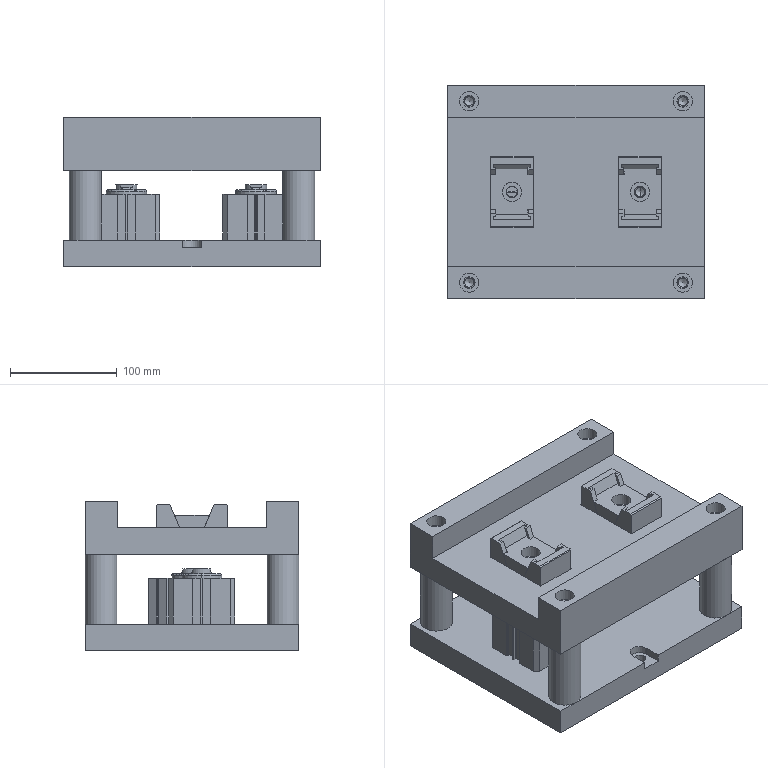Assembly | NX | mm | 20 component files | 20 solids | 812 faces | box 240 x 200 x 140.25 mm | volume 3239706 mm3 | plane 398 | cylinder 278 | cone 132 | torus 4 | commonest cylinder face diameters 0.4 x100 10.5 x32 0.8 x20 6.647 x16 11 x12 18 x12 8.5 x8 0.6 x8
Bill of materials:
unnamed part 1 | 4 |  | Long prismatic block with a trapezoidal side profile: one sloped face, and small chamfers on two corners. A T-shaped slot runs the full length and opens through the bottom face, so the end section has two downward legs.
unnamed part 2 | 2 |  | Squarish extruded body with four corner through-holes that have chamfered or counterbored rims. One end face has a raised circular boss with a central bore, surrounded by a shallow annular recess. Narrow lengthwise slots run along the side faces, and a lobe with a hexagonal-like outline sticks out from one side.
unnamed part 3 | 1 |  | Rectangular plate with raised rails along two opposite edges, giving a U-shaped channel section. There is a through-hole at each of the four corners on the rails. Two smaller holes in the channel floor each sit beside a shallow L-shaped scored line.
unnamed part 4 | 4 |  | Plain solid cylinder with a small coaxial hole in one end face, with a chamfered or countersunk entry.
unnamed part 5 | 2 |  | Stepped cylinder: a large short disc base with a smaller coaxial shaft on top. The upper part of the shaft has two opposite flats (double-D), and the shaft has a central bore with a chamfered entry.
unnamed part 6 | 2 |  | Square block with a central round through-hole. Two opposite side faces are tapered, so the section is a trapezoid that is wider at the top. There are small rectangular notches near the four corners and a groove on at least one sloped face.
unnamed part 7 | 4 |  | Long, slim body with a rectangular section. A smaller round cylindrical tail extends from one end. Near the other end there is a small circular feature on a face, and that end has a stepped or keyed shape with a small projecting tab.
unnamed part 8 | 1 |  | Flat rectangular plate with six through-holes: four near the corners and two at the middle of opposite long edges. The two middle holes sit inside stepped, U-shaped edge notches or counterbores.
Mates:
1. concentric | support_post 1 edge | base_plate 1 edge
2. concentric | support_post 4 | base_plate 1 edge
3. concentric | support_post 2 | base_plate 1 edge
4. concentric | support_post 3 | base_plate 1 edge
5. touch align | slide_table_part 1 face | support_post 1 face
6. align lock | slide_table_part 1 edge | support_post 1 edge
7. touch align | moving_slider 2 face | slide_table_part 1 face
8. touch align | moving_slider 1 face | slide_table_part 1 face
9. align lock | moving_slider 2 edge | slide_table_part 1 edge
10. align lock | moving_slider 1 face | slide_table_part 1 face
11. touch align | clamp_slider 3 face | moving_slider 1 face
12. touch align | clamp_slider 1 face | moving_slider 1 face
13. touch align | clamp_slider 4 face | moving_slider 2 face
14. touch align | clamp_slider 2 face | moving_slider 2 face
15. touch align | clamp_slider 3 face | moving_slider 1 face
16. align lock | clamp_slider 3 edge | moving_slider 1 edge
17. touch align | clamp_slider 1 face | moving_slider 1 face
18. align lock | clamp_slider 1 edge | moving_slider 1 edge
19. touch align | clamp_slider 2 face | moving_slider 2 face
20. touch align | clamp_slider 4 face | moving_slider 2 face
21. align lock | clamp_slider 4 edge | moving_slider 2 edge
22. align lock | clamp_slider 2 edge | moving_slider 2 edge
23. touch align | air_cylinder 1 face | base_plate 1 face
24. touch align | air_cylinder 2 face | base_plate 1 face